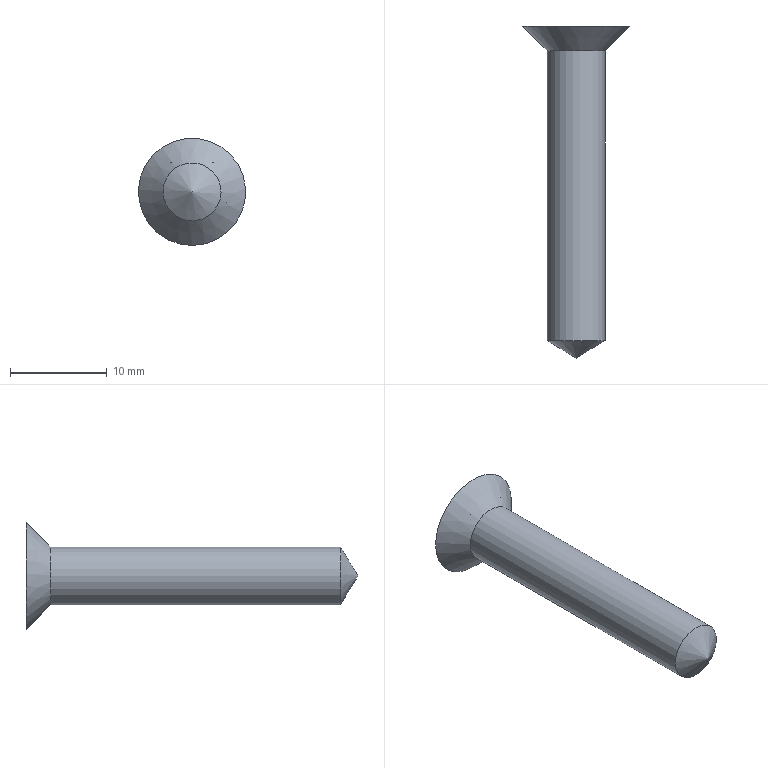Component | NX | SP_2SP1_2 | 1 solid | 10 faces | box 11.1 x 34.35 x 11.1 mm | volume 960 mm3 | plane 7 | cone 2 | cylinder 1 | commonest cylinder face diameters 6 x1
STEP:
#1=CARTESIAN_POINT('',(0.,0.,0.));
#2=DIRECTION('',(0.,0.,1.));
#3=DIRECTION('',(1.,0.,0.));
#4=AXIS2_PLACEMENT_3D('',#1,#2,#3);
#5=CARTESIAN_POINT('',(-108.104,120.,-12.399));
#6=VERTEX_POINT('',#5);
#7=CARTESIAN_POINT('',(-105.,120.,-17.));
#8=DIRECTION('',(0.,-1.,-0.));
#9=DIRECTION('',(-0.5592,-0.,0.829));
#10=AXIS2_PLACEMENT_3D('',#7,#8,#9);
#11=CIRCLE('',#10,5.55);
#12=CARTESIAN_POINT('',(-105.,120.,-17.));
#13=DIRECTION('',(0.,-1.,-0.));
#14=DIRECTION('',(-0.5592,-0.,0.829));
#15=AXIS2_PLACEMENT_3D('',#12,#13,#14);
#16=PLANE('',#15);
#17=CARTESIAN_POINT('',(0.,-0.));
#18=DIRECTION('',(1.,0.));
#19=AXIS2_PLACEMENT_2D('',#17,#18);
#20=CIRCLE('',#19,5.55);
#21=(GEOMETRIC_REPRESENTATION_CONTEXT(2)PARAMETRIC_REPRESENTATION_CONTEXT()REPRESENTATION_CONTEXT('',''));
#22=DEFINITIONAL_REPRESENTATION('',(#20),#21);
#23=PCURVE('',#16,#22);
#24=CARTESIAN_POINT('',(-105.,120.,-17.));
#25=DIRECTION('',(-0.,1.,0.));
#26=DIRECTION('',(0.5592,0.,-0.829));
#27=AXIS2_PLACEMENT_3D('',#24,#25,#26);
#28=CONICAL_SURFACE('',#27,5.55,0.7854);
#29=CARTESIAN_POINT('',(9.425,0.));
#30=DIRECTION('',(-1.,0.));
#31=VECTOR('',#30,1.);
#32=LINE('',#29,#31);
#33=(GEOMETRIC_REPRESENTATION_CONTEXT(2)PARAMETRIC_REPRESENTATION_CONTEXT()REPRESENTATION_CONTEXT('',''));
#34=DEFINITIONAL_REPRESENTATION('',(#32),#33);
#35=PCURVE('',#28,#34);
#36=SURFACE_CURVE('',#11,(#23,#35),.PCURVE_S1.);
#37=EDGE_CURVE('',#6,#6,#36,.T.);
#38=ORIENTED_EDGE('',*,*,#37,.F.);
#39=EDGE_LOOP('',(#38));
#40=FACE_BOUND('',#39,.T.);
#41=CARTESIAN_POINT('',(-102.82,120.,-14.));
#42=VERTEX_POINT('',#41);
#43=CARTESIAN_POINT('',(-101.473,120.,-18.146));
#44=VERTEX_POINT('',#43);
#45=CARTESIAN_POINT('',(-102.82,120.,-14.));
#46=DIRECTION('',(0.309,0.,-0.9511));
#47=VECTOR('',#46,1.);
#48=LINE('',#45,#47);
#49=CARTESIAN_POINT('',(1.268,-3.485));
#50=DIRECTION('',(-0.9613,0.2756));
#51=VECTOR('',#50,1.);
#52=LINE('',#49,#51);
#53=(GEOMETRIC_REPRESENTATION_CONTEXT(2)PARAMETRIC_REPRESENTATION_CONTEXT()REPRESENTATION_CONTEXT('',''));
#54=DEFINITIONAL_REPRESENTATION('',(#52),#53);
#55=PCURVE('',#16,#54);
#56=CARTESIAN_POINT('',(-102.82,118.3,-14.));
#57=DIRECTION('',(0.9511,0.,0.309));
#58=DIRECTION('',(-0.309,0.,0.9511));
#59=AXIS2_PLACEMENT_3D('',#56,#57,#58);
#60=PLANE('',#59);
#61=CARTESIAN_POINT('',(0.,-1.7));
#62=DIRECTION('',(-1.,0.));
#63=VECTOR('',#62,1.);
#64=LINE('',#61,#63);
#65=(GEOMETRIC_REPRESENTATION_CONTEXT(2)PARAMETRIC_REPRESENTATION_CONTEXT()REPRESENTATION_CONTEXT('',''));
#66=DEFINITIONAL_REPRESENTATION('',(#64),#65);
#67=PCURVE('',#60,#66);
#68=SURFACE_CURVE('',#48,(#55,#67),.PCURVE_S1.);
#69=EDGE_CURVE('',#42,#44,#68,.T.);
#70=ORIENTED_EDGE('',*,*,#69,.F.);
#71=CARTESIAN_POINT('',(-107.18,120.,-14.));
#72=VERTEX_POINT('',#71);
#73=CARTESIAN_POINT('',(-107.18,120.,-14.));
#74=DIRECTION('',(1.,0.,-0.));
#75=VECTOR('',#74,1.);
#76=LINE('',#73,#75);
#77=CARTESIAN_POINT('',(3.706,0.1294));
#78=DIRECTION('',(-0.5592,-0.829));
#79=VECTOR('',#78,1.);
#80=LINE('',#77,#79);
#81=(GEOMETRIC_REPRESENTATION_CONTEXT(2)PARAMETRIC_REPRESENTATION_CONTEXT()REPRESENTATION_CONTEXT('',''));
#82=DEFINITIONAL_REPRESENTATION('',(#80),#81);
#83=PCURVE('',#16,#82);
#84=CARTESIAN_POINT('',(-107.18,118.3,-14.));
#85=DIRECTION('',(0.,0.,1.));
#86=DIRECTION('',(-1.,0.,0.));
#87=AXIS2_PLACEMENT_3D('',#84,#85,#86);
#88=PLANE('',#87);
#89=CARTESIAN_POINT('',(0.,-1.7));
#90=DIRECTION('',(-1.,0.));
#91=VECTOR('',#90,1.);
#92=LINE('',#89,#91);
#93=(GEOMETRIC_REPRESENTATION_CONTEXT(2)PARAMETRIC_REPRESENTATION_CONTEXT()REPRESENTATION_CONTEXT('',''));
#94=DEFINITIONAL_REPRESENTATION('',(#92),#93);
#95=PCURVE('',#88,#94);
#96=SURFACE_CURVE('',#76,(#83,#95),.PCURVE_S1.);
#97=EDGE_CURVE('',#72,#42,#96,.T.);
#98=ORIENTED_EDGE('',*,*,#97,.F.);
#99=CARTESIAN_POINT('',(-108.527,120.,-18.146));
#100=VERTEX_POINT('',#99);
#101=CARTESIAN_POINT('',(-108.527,120.,-18.146));
#102=DIRECTION('',(0.309,0.,0.9511));
#103=VECTOR('',#102,1.);
#104=LINE('',#101,#103);
#105=CARTESIAN_POINT('',(1.022,3.565));
#106=DIRECTION('',(0.6157,-0.788));
#107=VECTOR('',#106,1.);
#108=LINE('',#105,#107);
#109=(GEOMETRIC_REPRESENTATION_CONTEXT(2)PARAMETRIC_REPRESENTATION_CONTEXT()REPRESENTATION_CONTEXT('',''));
#110=DEFINITIONAL_REPRESENTATION('',(#108),#109);
#111=PCURVE('',#16,#110);
#112=CARTESIAN_POINT('',(-108.527,118.3,-18.146));
#113=DIRECTION('',(-0.9511,0.,0.309));
#114=DIRECTION('',(-0.309,0.,-0.9511));
#115=AXIS2_PLACEMENT_3D('',#112,#113,#114);
#116=PLANE('',#115);
#117=CARTESIAN_POINT('',(0.,-1.7));
#118=DIRECTION('',(-1.,0.));
#119=VECTOR('',#118,1.);
#120=LINE('',#117,#119);
#121=(GEOMETRIC_REPRESENTATION_CONTEXT(2)PARAMETRIC_REPRESENTATION_CONTEXT()REPRESENTATION_CONTEXT('',''));
#122=DEFINITIONAL_REPRESENTATION('',(#120),#121);
#123=PCURVE('',#116,#122);
#124=SURFACE_CURVE('',#104,(#111,#123),.PCURVE_S1.);
#125=EDGE_CURVE('',#100,#72,#124,.T.);
#126=ORIENTED_EDGE('',*,*,#125,.F.);
#127=CARTESIAN_POINT('',(-105.,120.,-20.708));
#128=VERTEX_POINT('',#127);
#129=CARTESIAN_POINT('',(-105.,120.,-20.708));
#130=DIRECTION('',(-0.809,0.,0.5878));
#131=VECTOR('',#130,1.);
#132=LINE('',#129,#131);
#133=CARTESIAN_POINT('',(-3.074,2.074));
#134=DIRECTION('',(0.9397,0.342));
#135=VECTOR('',#134,1.);
#136=LINE('',#133,#135);
#137=(GEOMETRIC_REPRESENTATION_CONTEXT(2)PARAMETRIC_REPRESENTATION_CONTEXT()REPRESENTATION_CONTEXT('',''));
#138=DEFINITIONAL_REPRESENTATION('',(#136),#137);
#139=PCURVE('',#16,#138);
#140=CARTESIAN_POINT('',(-105.,118.3,-20.708));
#141=DIRECTION('',(-0.5878,0.,-0.809));
#142=DIRECTION('',(0.809,0.,-0.5878));
#143=AXIS2_PLACEMENT_3D('',#140,#141,#142);
#144=PLANE('',#143);
#145=CARTESIAN_POINT('',(0.,-1.7));
#146=DIRECTION('',(-1.,0.));
#147=VECTOR('',#146,1.);
#148=LINE('',#145,#147);
#149=(GEOMETRIC_REPRESENTATION_CONTEXT(2)PARAMETRIC_REPRESENTATION_CONTEXT()REPRESENTATION_CONTEXT('',''));
#150=DEFINITIONAL_REPRESENTATION('',(#148),#149);
#151=PCURVE('',#144,#150);
#152=SURFACE_CURVE('',#132,(#139,#151),.PCURVE_S1.);
#153=EDGE_CURVE('',#128,#100,#152,.T.);
#154=ORIENTED_EDGE('',*,*,#153,.F.);
#155=CARTESIAN_POINT('',(-101.473,120.,-18.146));
#156=DIRECTION('',(-0.809,0.,-0.5878));
#157=VECTOR('',#156,1.);
#158=LINE('',#155,#157);
#159=CARTESIAN_POINT('',(-2.922,-2.283));
#160=DIRECTION('',(-0.0349,0.9994));
#161=VECTOR('',#160,1.);
#162=LINE('',#159,#161);
#163=(GEOMETRIC_REPRESENTATION_CONTEXT(2)PARAMETRIC_REPRESENTATION_CONTEXT()REPRESENTATION_CONTEXT('',''));
#164=DEFINITIONAL_REPRESENTATION('',(#162),#163);
#165=PCURVE('',#16,#164);
#166=CARTESIAN_POINT('',(-101.473,118.3,-18.146));
#167=DIRECTION('',(0.5878,0.,-0.809));
#168=DIRECTION('',(0.809,0.,0.5878));
#169=AXIS2_PLACEMENT_3D('',#166,#167,#168);
#170=PLANE('',#169);
#171=CARTESIAN_POINT('',(0.,-1.7));
#172=DIRECTION('',(-1.,0.));
#173=VECTOR('',#172,1.);
#174=LINE('',#171,#173);
#175=(GEOMETRIC_REPRESENTATION_CONTEXT(2)PARAMETRIC_REPRESENTATION_CONTEXT()REPRESENTATION_CONTEXT('',''));
#176=DEFINITIONAL_REPRESENTATION('',(#174),#175);
#177=PCURVE('',#170,#176);
#178=SURFACE_CURVE('',#158,(#165,#177),.PCURVE_S1.);
#179=EDGE_CURVE('',#44,#128,#178,.T.);
#180=ORIENTED_EDGE('',*,*,#179,.F.);
#181=EDGE_LOOP('',(#70,#98,#126,#154,#180));
#182=FACE_BOUND('',#181,.T.);
#183=ADVANCED_FACE('',(#40,#182),#16,.F.);
#184=CARTESIAN_POINT('',(-106.678,117.45,-14.513));
#185=VERTEX_POINT('',#184);
#186=CARTESIAN_POINT('',(-105.,117.45,-17.));
#187=DIRECTION('',(0.,-1.,-0.));
#188=DIRECTION('',(-0.5592,-0.,0.829));
#189=AXIS2_PLACEMENT_3D('',#186,#187,#188);
#190=CIRCLE('',#189,3.);
#191=CARTESIAN_POINT('',(9.425,-2.55));
#192=DIRECTION('',(-1.,0.));
#193=VECTOR('',#192,1.);
#194=LINE('',#191,#193);
#195=(GEOMETRIC_REPRESENTATION_CONTEXT(2)PARAMETRIC_REPRESENTATION_CONTEXT()REPRESENTATION_CONTEXT('',''));
#196=DEFINITIONAL_REPRESENTATION('',(#194),#195);
#197=PCURVE('',#28,#196);
#198=CARTESIAN_POINT('',(-105.,120.,-17.));
#199=DIRECTION('',(0.,-1.,-0.));
#200=DIRECTION('',(-0.5592,-0.,0.829));
#201=AXIS2_PLACEMENT_3D('',#198,#199,#200);
#202=CYLINDRICAL_SURFACE('',#201,3.);
#203=CARTESIAN_POINT('',(0.,2.55));
#204=DIRECTION('',(1.,0.));
#205=VECTOR('',#204,1.);
#206=LINE('',#203,#205);
#207=(GEOMETRIC_REPRESENTATION_CONTEXT(2)PARAMETRIC_REPRESENTATION_CONTEXT()REPRESENTATION_CONTEXT('',''));
#208=DEFINITIONAL_REPRESENTATION('',(#206),#207);
#209=PCURVE('',#202,#208);
#210=SURFACE_CURVE('',#190,(#197,#209),.PCURVE_S1.);
#211=EDGE_CURVE('',#185,#185,#210,.T.);
#212=ORIENTED_EDGE('',*,*,#211,.F.);
#213=CARTESIAN_POINT('',(-106.678,117.45,-14.513));
#214=CARTESIAN_POINT('',(-108.104,120.,-12.399));
#215=B_SPLINE_CURVE_WITH_KNOTS('',1,(#213,#214),.UNSPECIFIED.,.F.,.F.,(2,2),(-3.606,0.),.PIECEWISE_BEZIER_KNOTS.);
#216=CARTESIAN_POINT('',(9.425,0.));
#217=DIRECTION('',(0.,1.));
#218=VECTOR('',#217,1.);
#219=LINE('',#216,#218);
#220=(GEOMETRIC_REPRESENTATION_CONTEXT(2)PARAMETRIC_REPRESENTATION_CONTEXT()REPRESENTATION_CONTEXT('',''));
#221=DEFINITIONAL_REPRESENTATION('',(#219),#220);
#222=PCURVE('',#28,#221);
#223=CARTESIAN_POINT('',(3.142,0.));
#224=DIRECTION('',(0.,1.));
#225=VECTOR('',#224,1.);
#226=LINE('',#223,#225);
#227=(GEOMETRIC_REPRESENTATION_CONTEXT(2)PARAMETRIC_REPRESENTATION_CONTEXT()REPRESENTATION_CONTEXT('',''));
#228=DEFINITIONAL_REPRESENTATION('',(#226),#227);
#229=PCURVE('',#28,#228);
#230=SEAM_CURVE('',#215,(#222,#229),.PCURVE_S1.);
#231=EDGE_CURVE('',#185,#6,#230,.T.);
#232=ORIENTED_EDGE('',*,*,#231,.T.);
#233=ORIENTED_EDGE('',*,*,#37,.T.);
#234=ORIENTED_EDGE('',*,*,#231,.F.);
#235=EDGE_LOOP('',(#212,#232,#233,#234));
#236=FACE_BOUND('',#235,.T.);
#237=ADVANCED_FACE('',(#236),#28,.T.);
#238=CARTESIAN_POINT('',(-106.678,87.45,-14.513));
#239=VERTEX_POINT('',#238);
#240=CARTESIAN_POINT('',(-103.322,87.45,-19.487));
#241=VERTEX_POINT('',#240);
#242=CARTESIAN_POINT('',(-105.,87.45,-17.));
#243=DIRECTION('',(0.,-1.,-0.));
#244=DIRECTION('',(-0.5592,-0.,0.829));
#245=AXIS2_PLACEMENT_3D('',#242,#243,#244);
#246=CIRCLE('',#245,3.);
#247=CARTESIAN_POINT('',(0.,32.55));
#248=DIRECTION('',(1.,0.));
#249=VECTOR('',#248,1.);
#250=LINE('',#247,#249);
#251=(GEOMETRIC_REPRESENTATION_CONTEXT(2)PARAMETRIC_REPRESENTATION_CONTEXT()REPRESENTATION_CONTEXT('',''));
#252=DEFINITIONAL_REPRESENTATION('',(#250),#251);
#253=PCURVE('',#202,#252);
#254=CARTESIAN_POINT('',(-105.,87.45,-17.));
#255=DIRECTION('',(-0.,1.,0.));
#256=DIRECTION('',(0.5592,0.,-0.829));
#257=AXIS2_PLACEMENT_3D('',#254,#255,#256);
#258=CONICAL_SURFACE('',#257,3.,1.03);
#259=CARTESIAN_POINT('',(3.142,0.));
#260=DIRECTION('',(-1.,0.));
#261=VECTOR('',#260,1.);
#262=LINE('',#259,#261);
#263=(GEOMETRIC_REPRESENTATION_CONTEXT(2)PARAMETRIC_REPRESENTATION_CONTEXT()REPRESENTATION_CONTEXT('',''));
#264=DEFINITIONAL_REPRESENTATION('',(#262),#263);
#265=PCURVE('',#258,#264);
#266=SURFACE_CURVE('',#246,(#253,#265),.PCURVE_S1.);
#267=EDGE_CURVE('',#239,#241,#266,.T.);
#268=ORIENTED_EDGE('',*,*,#267,.F.);
#269=CARTESIAN_POINT('',(-106.678,117.45,-14.513));
#270=CARTESIAN_POINT('',(-106.678,87.45,-14.513));
#271=B_SPLINE_CURVE_WITH_KNOTS('',1,(#269,#270),.UNSPECIFIED.,.F.,.F.,(2,2),(2.55,32.55),.PIECEWISE_BEZIER_KNOTS.);
#272=CARTESIAN_POINT('',(0.,0.));
#273=DIRECTION('',(0.,1.));
#274=VECTOR('',#273,1.);
#275=LINE('',#272,#274);
#276=(GEOMETRIC_REPRESENTATION_CONTEXT(2)PARAMETRIC_REPRESENTATION_CONTEXT()REPRESENTATION_CONTEXT('',''));
#277=DEFINITIONAL_REPRESENTATION('',(#275),#276);
#278=PCURVE('',#202,#277);
#279=CARTESIAN_POINT('',(6.283,0.));
#280=DIRECTION('',(0.,1.));
#281=VECTOR('',#280,1.);
#282=LINE('',#279,#281);
#283=(GEOMETRIC_REPRESENTATION_CONTEXT(2)PARAMETRIC_REPRESENTATION_CONTEXT()REPRESENTATION_CONTEXT('',''));
#284=DEFINITIONAL_REPRESENTATION('',(#282),#283);
#285=PCURVE('',#202,#284);
#286=SEAM_CURVE('',#271,(#278,#285),.PCURVE_S1.);
#287=EDGE_CURVE('',#185,#239,#286,.T.);
#288=ORIENTED_EDGE('',*,*,#287,.F.);
#289=ORIENTED_EDGE('',*,*,#211,.T.);
#290=ORIENTED_EDGE('',*,*,#287,.T.);
#291=CARTESIAN_POINT('',(-105.,87.45,-17.));
#292=DIRECTION('',(0.,-1.,-0.));
#293=DIRECTION('',(-0.5592,-0.,0.829));
#294=AXIS2_PLACEMENT_3D('',#291,#292,#293);
#295=CIRCLE('',#294,3.);
#296=CARTESIAN_POINT('',(0.,32.55));
#297=DIRECTION('',(1.,0.));
#298=VECTOR('',#297,1.);
#299=LINE('',#296,#298);
#300=(GEOMETRIC_REPRESENTATION_CONTEXT(2)PARAMETRIC_REPRESENTATION_CONTEXT()REPRESENTATION_CONTEXT('',''));
#301=DEFINITIONAL_REPRESENTATION('',(#299),#300);
#302=PCURVE('',#202,#301);
#303=CARTESIAN_POINT('',(9.425,0.));
#304=DIRECTION('',(-1.,0.));
#305=VECTOR('',#304,1.);
#306=LINE('',#303,#305);
#307=(GEOMETRIC_REPRESENTATION_CONTEXT(2)PARAMETRIC_REPRESENTATION_CONTEXT()REPRESENTATION_CONTEXT('',''));
#308=DEFINITIONAL_REPRESENTATION('',(#306),#307);
#309=PCURVE('',#258,#308);
#310=SURFACE_CURVE('',#295,(#302,#309),.PCURVE_S1.);
#311=EDGE_CURVE('',#241,#239,#310,.T.);
#312=ORIENTED_EDGE('',*,*,#311,.F.);
#313=EDGE_LOOP('',(#268,#288,#289,#290,#312));
#314=FACE_BOUND('',#313,.T.);
#315=ADVANCED_FACE('',(#314),#202,.T.);
#316=CARTESIAN_POINT('',(-105.,85.647,-17.));
#317=VERTEX_POINT('',#316);
#318=CARTESIAN_POINT('',(-105.,85.647,-17.));
#319=CARTESIAN_POINT('',(-103.322,87.45,-19.487));
#320=B_SPLINE_CURVE_WITH_KNOTS('',1,(#318,#319),.UNSPECIFIED.,.F.,.F.,(2,2),(-3.5,0.),.PIECEWISE_BEZIER_KNOTS.);
#321=CARTESIAN_POINT('',(6.283,0.));
#322=DIRECTION('',(0.,1.));
#323=VECTOR('',#322,1.);
#324=LINE('',#321,#323);
#325=(GEOMETRIC_REPRESENTATION_CONTEXT(2)PARAMETRIC_REPRESENTATION_CONTEXT()REPRESENTATION_CONTEXT('',''));
#326=DEFINITIONAL_REPRESENTATION('',(#324),#325);
#327=PCURVE('',#258,#326);
#328=CARTESIAN_POINT('',(0.,0.));
#329=DIRECTION('',(0.,1.));
#330=VECTOR('',#329,1.);
#331=LINE('',#328,#330);
#332=(GEOMETRIC_REPRESENTATION_CONTEXT(2)PARAMETRIC_REPRESENTATION_CONTEXT()REPRESENTATION_CONTEXT('',''));
#333=DEFINITIONAL_REPRESENTATION('',(#331),#332);
#334=PCURVE('',#258,#333);
#335=SEAM_CURVE('',#320,(#327,#334),.PCURVE_S1.);
#336=EDGE_CURVE('',#317,#241,#335,.T.);
#337=ORIENTED_EDGE('',*,*,#336,.T.);
#338=ORIENTED_EDGE('',*,*,#311,.T.);
#339=ORIENTED_EDGE('',*,*,#267,.T.);
#340=ORIENTED_EDGE('',*,*,#336,.F.);
#341=EDGE_LOOP('',(#337,#338,#339,#340));
#342=FACE_BOUND('',#341,.T.);
#343=ADVANCED_FACE('',(#342),#258,.T.);
#344=ORIENTED_EDGE('',*,*,#69,.T.);
#345=CARTESIAN_POINT('',(-101.473,118.3,-18.146));
#346=VERTEX_POINT('',#345);
#347=CARTESIAN_POINT('',(-101.473,118.3,-18.146));
#348=DIRECTION('',(0.,-1.,0.));
#349=VECTOR('',#348,1.);
#350=LINE('',#347,#349);
#351=CARTESIAN_POINT('',(-4.359,0.));
#352=DIRECTION('',(0.,1.));
#353=VECTOR('',#352,1.);
#354=LINE('',#351,#353);
#355=(GEOMETRIC_REPRESENTATION_CONTEXT(2)PARAMETRIC_REPRESENTATION_CONTEXT()REPRESENTATION_CONTEXT('',''));
#356=DEFINITIONAL_REPRESENTATION('',(#354),#355);
#357=PCURVE('',#60,#356);
#358=CARTESIAN_POINT('',(0.,0.));
#359=DIRECTION('',(0.,1.));
#360=VECTOR('',#359,1.);
#361=LINE('',#358,#360);
#362=(GEOMETRIC_REPRESENTATION_CONTEXT(2)PARAMETRIC_REPRESENTATION_CONTEXT()REPRESENTATION_CONTEXT('',''));
#363=DEFINITIONAL_REPRESENTATION('',(#361),#362);
#364=PCURVE('',#170,#363);
#365=SURFACE_CURVE('',#350,(#357,#364),.PCURVE_S1.);
#366=EDGE_CURVE('',#44,#346,#365,.T.);
#367=ORIENTED_EDGE('',*,*,#366,.T.);
#368=CARTESIAN_POINT('',(-102.82,118.3,-14.));
#369=VERTEX_POINT('',#368);
#370=CARTESIAN_POINT('',(-102.82,118.3,-14.));
#371=DIRECTION('',(-0.309,0.,0.9511));
#372=VECTOR('',#371,1.);
#373=LINE('',#370,#372);
#374=CARTESIAN_POINT('',(0.,0.));
#375=DIRECTION('',(1.,0.));
#376=VECTOR('',#375,1.);
#377=LINE('',#374,#376);
#378=(GEOMETRIC_REPRESENTATION_CONTEXT(2)PARAMETRIC_REPRESENTATION_CONTEXT()REPRESENTATION_CONTEXT('',''));
#379=DEFINITIONAL_REPRESENTATION('',(#377),#378);
#380=PCURVE('',#60,#379);
#381=CARTESIAN_POINT('',(-105.,118.3,-17.));
#382=DIRECTION('',(0.,1.,0.));
#383=DIRECTION('',(0.829,0.,0.5592));
#384=AXIS2_PLACEMENT_3D('',#381,#382,#383);
#385=PLANE('',#384);
#386=CARTESIAN_POINT('',(3.485,-1.268));
#387=DIRECTION('',(0.2756,-0.9613));
#388=VECTOR('',#387,1.);
#389=LINE('',#386,#388);
#390=(GEOMETRIC_REPRESENTATION_CONTEXT(2)PARAMETRIC_REPRESENTATION_CONTEXT()REPRESENTATION_CONTEXT('',''));
#391=DEFINITIONAL_REPRESENTATION('',(#389),#390);
#392=PCURVE('',#385,#391);
#393=SURFACE_CURVE('',#373,(#380,#392),.PCURVE_S1.);
#394=EDGE_CURVE('',#346,#369,#393,.T.);
#395=ORIENTED_EDGE('',*,*,#394,.T.);
#396=CARTESIAN_POINT('',(-102.82,118.3,-14.));
#397=DIRECTION('',(0.,-1.,0.));
#398=VECTOR('',#397,1.);
#399=LINE('',#396,#398);
#400=CARTESIAN_POINT('',(0.,0.));
#401=DIRECTION('',(0.,1.));
#402=VECTOR('',#401,1.);
#403=LINE('',#400,#402);
#404=(GEOMETRIC_REPRESENTATION_CONTEXT(2)PARAMETRIC_REPRESENTATION_CONTEXT()REPRESENTATION_CONTEXT('',''));
#405=DEFINITIONAL_REPRESENTATION('',(#403),#404);
#406=PCURVE('',#60,#405);
#407=CARTESIAN_POINT('',(-4.359,0.));
#408=DIRECTION('',(0.,1.));
#409=VECTOR('',#408,1.);
#410=LINE('',#407,#409);
#411=(GEOMETRIC_REPRESENTATION_CONTEXT(2)PARAMETRIC_REPRESENTATION_CONTEXT()REPRESENTATION_CONTEXT('',''));
#412=DEFINITIONAL_REPRESENTATION('',(#410),#411);
#413=PCURVE('',#88,#412);
#414=SURFACE_CURVE('',#399,(#406,#413),.PCURVE_S1.);
#415=EDGE_CURVE('',#42,#369,#414,.T.);
#416=ORIENTED_EDGE('',*,*,#415,.F.);
#417=EDGE_LOOP('',(#344,#367,#395,#416));
#418=FACE_BOUND('',#417,.T.);
#419=ADVANCED_FACE('',(#418),#60,.F.);
#420=ORIENTED_EDGE('',*,*,#179,.T.);
#421=CARTESIAN_POINT('',(-105.,118.3,-20.708));
#422=VERTEX_POINT('',#421);
#423=CARTESIAN_POINT('',(-105.,118.3,-20.708));
#424=DIRECTION('',(0.,-1.,0.));
#425=VECTOR('',#424,1.);
#426=LINE('',#423,#425);
#427=CARTESIAN_POINT('',(-4.359,0.));
#428=DIRECTION('',(0.,1.));
#429=VECTOR('',#428,1.);
#430=LINE('',#427,#429);
#431=(GEOMETRIC_REPRESENTATION_CONTEXT(2)PARAMETRIC_REPRESENTATION_CONTEXT()REPRESENTATION_CONTEXT('',''));
#432=DEFINITIONAL_REPRESENTATION('',(#430),#431);
#433=PCURVE('',#170,#432);
#434=CARTESIAN_POINT('',(0.,0.));
#435=DIRECTION('',(0.,1.));
#436=VECTOR('',#435,1.);
#437=LINE('',#434,#436);
#438=(GEOMETRIC_REPRESENTATION_CONTEXT(2)PARAMETRIC_REPRESENTATION_CONTEXT()REPRESENTATION_CONTEXT('',''));
#439=DEFINITIONAL_REPRESENTATION('',(#437),#438);
#440=PCURVE('',#144,#439);
#441=SURFACE_CURVE('',#426,(#433,#440),.PCURVE_S1.);
#442=EDGE_CURVE('',#128,#422,#441,.T.);
#443=ORIENTED_EDGE('',*,*,#442,.T.);
#444=CARTESIAN_POINT('',(-101.473,118.3,-18.146));
#445=DIRECTION('',(0.809,0.,0.5878));
#446=VECTOR('',#445,1.);
#447=LINE('',#444,#446);
#448=CARTESIAN_POINT('',(0.,0.));
#449=DIRECTION('',(1.,0.));
#450=VECTOR('',#449,1.);
#451=LINE('',#448,#450);
#452=(GEOMETRIC_REPRESENTATION_CONTEXT(2)PARAMETRIC_REPRESENTATION_CONTEXT()REPRESENTATION_CONTEXT('',''));
#453=DEFINITIONAL_REPRESENTATION('',(#451),#452);
#454=PCURVE('',#170,#453);
#455=CARTESIAN_POINT('',(2.283,2.922));
#456=DIRECTION('',(0.9994,-0.0349));
#457=VECTOR('',#456,1.);
#458=LINE('',#455,#457);
#459=(GEOMETRIC_REPRESENTATION_CONTEXT(2)PARAMETRIC_REPRESENTATION_CONTEXT()REPRESENTATION_CONTEXT('',''));
#460=DEFINITIONAL_REPRESENTATION('',(#458),#459);
#461=PCURVE('',#385,#460);
#462=SURFACE_CURVE('',#447,(#454,#461),.PCURVE_S1.);
#463=EDGE_CURVE('',#422,#346,#462,.T.);
#464=ORIENTED_EDGE('',*,*,#463,.T.);
#465=ORIENTED_EDGE('',*,*,#366,.F.);
#466=EDGE_LOOP('',(#420,#443,#464,#465));
#467=FACE_BOUND('',#466,.T.);
#468=ADVANCED_FACE('',(#467),#170,.F.);
#469=ORIENTED_EDGE('',*,*,#153,.T.);
#470=CARTESIAN_POINT('',(-108.527,118.3,-18.146));
#471=VERTEX_POINT('',#470);
#472=CARTESIAN_POINT('',(-108.527,118.3,-18.146));
#473=DIRECTION('',(0.,-1.,0.));
#474=VECTOR('',#473,1.);
#475=LINE('',#472,#474);
#476=CARTESIAN_POINT('',(-4.359,0.));
#477=DIRECTION('',(0.,1.));
#478=VECTOR('',#477,1.);
#479=LINE('',#476,#478);
#480=(GEOMETRIC_REPRESENTATION_CONTEXT(2)PARAMETRIC_REPRESENTATION_CONTEXT()REPRESENTATION_CONTEXT('',''));
#481=DEFINITIONAL_REPRESENTATION('',(#479),#480);
#482=PCURVE('',#144,#481);
#483=CARTESIAN_POINT('',(0.,0.));
#484=DIRECTION('',(0.,1.));
#485=VECTOR('',#484,1.);
#486=LINE('',#483,#485);
#487=(GEOMETRIC_REPRESENTATION_CONTEXT(2)PARAMETRIC_REPRESENTATION_CONTEXT()REPRESENTATION_CONTEXT('',''));
#488=DEFINITIONAL_REPRESENTATION('',(#486),#487);
#489=PCURVE('',#116,#488);
#490=SURFACE_CURVE('',#475,(#482,#489),.PCURVE_S1.);
#491=EDGE_CURVE('',#100,#471,#490,.T.);
#492=ORIENTED_EDGE('',*,*,#491,.T.);
#493=CARTESIAN_POINT('',(-105.,118.3,-20.708));
#494=DIRECTION('',(0.809,0.,-0.5878));
#495=VECTOR('',#494,1.);
#496=LINE('',#493,#495);
#497=CARTESIAN_POINT('',(0.,0.));
#498=DIRECTION('',(1.,0.));
#499=VECTOR('',#498,1.);
#500=LINE('',#497,#499);
#501=(GEOMETRIC_REPRESENTATION_CONTEXT(2)PARAMETRIC_REPRESENTATION_CONTEXT()REPRESENTATION_CONTEXT('',''));
#502=DEFINITIONAL_REPRESENTATION('',(#500),#501);
#503=PCURVE('',#144,#502);
#504=CARTESIAN_POINT('',(-2.074,3.074));
#505=DIRECTION('',(0.342,0.9397));
#506=VECTOR('',#505,1.);
#507=LINE('',#504,#506);
#508=(GEOMETRIC_REPRESENTATION_CONTEXT(2)PARAMETRIC_REPRESENTATION_CONTEXT()REPRESENTATION_CONTEXT('',''));
#509=DEFINITIONAL_REPRESENTATION('',(#507),#508);
#510=PCURVE('',#385,#509);
#511=SURFACE_CURVE('',#496,(#503,#510),.PCURVE_S1.);
#512=EDGE_CURVE('',#471,#422,#511,.T.);
#513=ORIENTED_EDGE('',*,*,#512,.T.);
#514=ORIENTED_EDGE('',*,*,#442,.F.);
#515=EDGE_LOOP('',(#469,#492,#513,#514));
#516=FACE_BOUND('',#515,.T.);
#517=ADVANCED_FACE('',(#516),#144,.F.);
#518=ORIENTED_EDGE('',*,*,#125,.T.);
#519=CARTESIAN_POINT('',(-107.18,118.3,-14.));
#520=VERTEX_POINT('',#519);
#521=CARTESIAN_POINT('',(-107.18,118.3,-14.));
#522=DIRECTION('',(0.,-1.,0.));
#523=VECTOR('',#522,1.);
#524=LINE('',#521,#523);
#525=CARTESIAN_POINT('',(-4.359,0.));
#526=DIRECTION('',(0.,1.));
#527=VECTOR('',#526,1.);
#528=LINE('',#525,#527);
#529=(GEOMETRIC_REPRESENTATION_CONTEXT(2)PARAMETRIC_REPRESENTATION_CONTEXT()REPRESENTATION_CONTEXT('',''));
#530=DEFINITIONAL_REPRESENTATION('',(#528),#529);
#531=PCURVE('',#116,#530);
#532=CARTESIAN_POINT('',(0.,0.));
#533=DIRECTION('',(0.,1.));
#534=VECTOR('',#533,1.);
#535=LINE('',#532,#534);
#536=(GEOMETRIC_REPRESENTATION_CONTEXT(2)PARAMETRIC_REPRESENTATION_CONTEXT()REPRESENTATION_CONTEXT('',''));
#537=DEFINITIONAL_REPRESENTATION('',(#535),#536);
#538=PCURVE('',#88,#537);
#539=SURFACE_CURVE('',#524,(#531,#538),.PCURVE_S1.);
#540=EDGE_CURVE('',#72,#520,#539,.T.);
#541=ORIENTED_EDGE('',*,*,#540,.T.);
#542=CARTESIAN_POINT('',(-108.527,118.3,-18.146));
#543=DIRECTION('',(-0.309,0.,-0.9511));
#544=VECTOR('',#543,1.);
#545=LINE('',#542,#544);
#546=CARTESIAN_POINT('',(0.,0.));
#547=DIRECTION('',(1.,0.));
#548=VECTOR('',#547,1.);
#549=LINE('',#546,#548);
#550=(GEOMETRIC_REPRESENTATION_CONTEXT(2)PARAMETRIC_REPRESENTATION_CONTEXT()REPRESENTATION_CONTEXT('',''));
#551=DEFINITIONAL_REPRESENTATION('',(#549),#550);
#552=PCURVE('',#116,#551);
#553=CARTESIAN_POINT('',(-3.565,-1.022));
#554=DIRECTION('',(-0.788,0.6157));
#555=VECTOR('',#554,1.);
#556=LINE('',#553,#555);
#557=(GEOMETRIC_REPRESENTATION_CONTEXT(2)PARAMETRIC_REPRESENTATION_CONTEXT()REPRESENTATION_CONTEXT('',''));
#558=DEFINITIONAL_REPRESENTATION('',(#556),#557);
#559=PCURVE('',#385,#558);
#560=SURFACE_CURVE('',#545,(#552,#559),.PCURVE_S1.);
#561=EDGE_CURVE('',#520,#471,#560,.T.);
#562=ORIENTED_EDGE('',*,*,#561,.T.);
#563=ORIENTED_EDGE('',*,*,#491,.F.);
#564=EDGE_LOOP('',(#518,#541,#562,#563));
#565=FACE_BOUND('',#564,.T.);
#566=ADVANCED_FACE('',(#565),#116,.F.);
#567=ORIENTED_EDGE('',*,*,#97,.T.);
#568=ORIENTED_EDGE('',*,*,#415,.T.);
#569=CARTESIAN_POINT('',(-107.18,118.3,-14.));
#570=DIRECTION('',(-1.,0.,0.));
#571=VECTOR('',#570,1.);
#572=LINE('',#569,#571);
#573=CARTESIAN_POINT('',(0.,0.));
#574=DIRECTION('',(1.,0.));
#575=VECTOR('',#574,1.);
#576=LINE('',#573,#575);
#577=(GEOMETRIC_REPRESENTATION_CONTEXT(2)PARAMETRIC_REPRESENTATION_CONTEXT()REPRESENTATION_CONTEXT('',''));
#578=DEFINITIONAL_REPRESENTATION('',(#576),#577);
#579=PCURVE('',#88,#578);
#580=CARTESIAN_POINT('',(-0.1294,-3.706));
#581=DIRECTION('',(-0.829,-0.5592));
#582=VECTOR('',#581,1.);
#583=LINE('',#580,#582);
#584=(GEOMETRIC_REPRESENTATION_CONTEXT(2)PARAMETRIC_REPRESENTATION_CONTEXT()REPRESENTATION_CONTEXT('',''));
#585=DEFINITIONAL_REPRESENTATION('',(#583),#584);
#586=PCURVE('',#385,#585);
#587=SURFACE_CURVE('',#572,(#579,#586),.PCURVE_S1.);
#588=EDGE_CURVE('',#369,#520,#587,.T.);
#589=ORIENTED_EDGE('',*,*,#588,.T.);
#590=ORIENTED_EDGE('',*,*,#540,.F.);
#591=EDGE_LOOP('',(#567,#568,#589,#590));
#592=FACE_BOUND('',#591,.T.);
#593=ADVANCED_FACE('',(#592),#88,.F.);
#594=ORIENTED_EDGE('',*,*,#394,.F.);
#595=ORIENTED_EDGE('',*,*,#463,.F.);
#596=ORIENTED_EDGE('',*,*,#512,.F.);
#597=ORIENTED_EDGE('',*,*,#561,.F.);
#598=ORIENTED_EDGE('',*,*,#588,.F.);
#599=EDGE_LOOP('',(#594,#595,#596,#597,#598));
#600=FACE_BOUND('',#599,.T.);
#601=ADVANCED_FACE('',(#600),#385,.T.);
#602=CLOSED_SHELL('',(#183,#237,#315,#343,#419,#468,#517,#566,#593,#601));
#603=MANIFOLD_SOLID_BREP('',#602);
#604=(LENGTH_UNIT()NAMED_UNIT(*)SI_UNIT(.MILLI.,.METRE.));
#605=UNCERTAINTY_MEASURE_WITH_UNIT(LENGTH_MEASURE(0.000002),#604,'','');
#606=(NAMED_UNIT(*)PLANE_ANGLE_UNIT()SI_UNIT($,.RADIAN.));
#607=(NAMED_UNIT(*)SI_UNIT($,.STERADIAN.)SOLID_ANGLE_UNIT());
#608=(GEOMETRIC_REPRESENTATION_CONTEXT(3)GLOBAL_UNCERTAINTY_ASSIGNED_CONTEXT((#605))GLOBAL_UNIT_ASSIGNED_CONTEXT((#604,#606,#607))REPRESENTATION_CONTEXT('',''));
#609=ADVANCED_BREP_SHAPE_REPRESENTATION('',(#4,#603),#608);